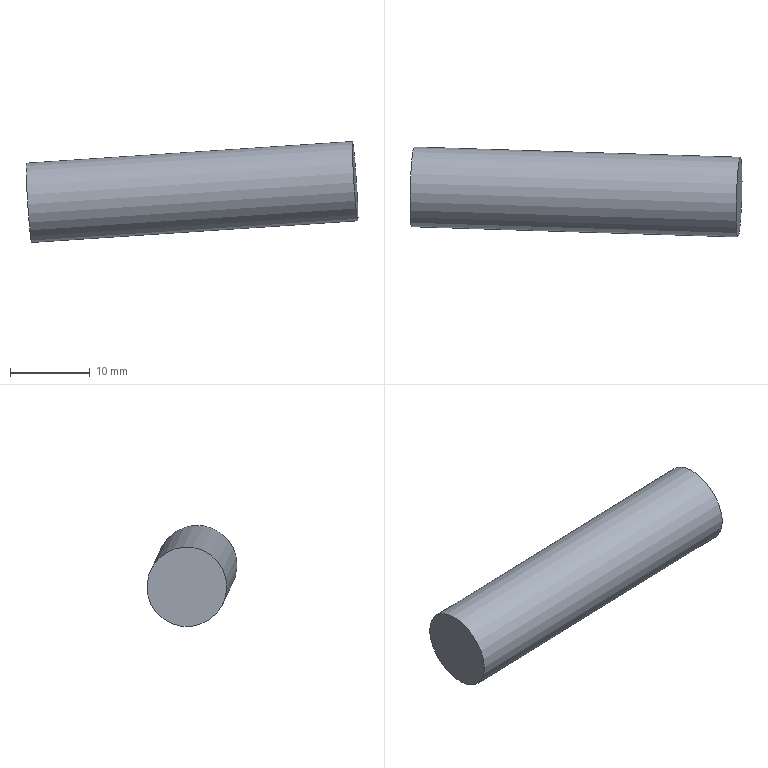Component | NX | KEY2 | 1 solid | 3 faces | box 41.62 x 11.28 x 12.69 mm | volume 3220 mm3 | plane 2 | cylinder 1 | commonest cylinder face diameters 10 x1
STEP:
#1=CARTESIAN_POINT('',(0.,0.,0.));
#2=DIRECTION('',(0.,0.,1.));
#3=DIRECTION('',(1.,0.,0.));
#4=AXIS2_PLACEMENT_3D('',#1,#2,#3);
#5=CARTESIAN_POINT('',(261.275,-324.256,279.125));
#6=VERTEX_POINT('',#5);
#7=CARTESIAN_POINT('',(261.248,-319.91,281.596));
#8=DIRECTION('',(-0.9973,0.03139,-0.06617));
#9=DIRECTION('',(0.005429,-0.8693,-0.4942));
#10=AXIS2_PLACEMENT_3D('',#7,#8,#9);
#11=CIRCLE('',#10,5.);
#12=CARTESIAN_POINT('',(261.248,-319.91,281.596));
#13=DIRECTION('',(0.9973,-0.03139,0.06617));
#14=DIRECTION('',(-0.07304,-0.4932,0.8668));
#15=AXIS2_PLACEMENT_3D('',#12,#13,#14);
#16=CYLINDRICAL_SURFACE('',#15,5.);
#17=CARTESIAN_POINT('',(7.854,0.));
#18=DIRECTION('',(-1.,0.));
#19=VECTOR('',#18,1.);
#20=LINE('',#17,#19);
#21=(GEOMETRIC_REPRESENTATION_CONTEXT(2)PARAMETRIC_REPRESENTATION_CONTEXT()REPRESENTATION_CONTEXT('',''));
#22=DEFINITIONAL_REPRESENTATION('',(#20),#21);
#23=PCURVE('',#16,#22);
#24=CARTESIAN_POINT('',(261.248,-319.91,281.596));
#25=DIRECTION('',(-0.9973,0.03139,-0.06617));
#26=DIRECTION('',(0.07304,0.4932,-0.8668));
#27=AXIS2_PLACEMENT_3D('',#24,#25,#26);
#28=PLANE('',#27);
#29=CARTESIAN_POINT('',(0.,0.));
#30=DIRECTION('',(-0.,1.));
#31=AXIS2_PLACEMENT_2D('',#29,#30);
#32=CIRCLE('',#31,5.);
#33=(GEOMETRIC_REPRESENTATION_CONTEXT(2)PARAMETRIC_REPRESENTATION_CONTEXT()REPRESENTATION_CONTEXT('',''));
#34=DEFINITIONAL_REPRESENTATION('',(#32),#33);
#35=PCURVE('',#28,#34);
#36=SURFACE_CURVE('',#11,(#23,#35),.PCURVE_S1.);
#37=EDGE_CURVE('',#6,#6,#36,.T.);
#38=ORIENTED_EDGE('',*,*,#37,.F.);
#39=CARTESIAN_POINT('',(302.165,-325.543,281.838));
#40=VERTEX_POINT('',#39);
#41=CARTESIAN_POINT('',(261.275,-324.256,279.125));
#42=CARTESIAN_POINT('',(302.165,-325.543,281.838));
#43=B_SPLINE_CURVE_WITH_KNOTS('',1,(#41,#42),.UNSPECIFIED.,.F.,.F.,(2,2),(0.,41.),.PIECEWISE_BEZIER_KNOTS.);
#44=CARTESIAN_POINT('',(7.854,0.));
#45=DIRECTION('',(0.,1.));
#46=VECTOR('',#45,1.);
#47=LINE('',#44,#46);
#48=(GEOMETRIC_REPRESENTATION_CONTEXT(2)PARAMETRIC_REPRESENTATION_CONTEXT()REPRESENTATION_CONTEXT('',''));
#49=DEFINITIONAL_REPRESENTATION('',(#47),#48);
#50=PCURVE('',#16,#49);
#51=CARTESIAN_POINT('',(1.571,0.));
#52=DIRECTION('',(0.,1.));
#53=VECTOR('',#52,1.);
#54=LINE('',#51,#53);
#55=(GEOMETRIC_REPRESENTATION_CONTEXT(2)PARAMETRIC_REPRESENTATION_CONTEXT()REPRESENTATION_CONTEXT('',''));
#56=DEFINITIONAL_REPRESENTATION('',(#54),#55);
#57=PCURVE('',#16,#56);
#58=SEAM_CURVE('',#43,(#50,#57),.PCURVE_S1.);
#59=EDGE_CURVE('',#6,#40,#58,.T.);
#60=ORIENTED_EDGE('',*,*,#59,.T.);
#61=CARTESIAN_POINT('',(302.138,-321.197,284.309));
#62=DIRECTION('',(-0.9973,0.03139,-0.06617));
#63=DIRECTION('',(0.005429,-0.8693,-0.4942));
#64=AXIS2_PLACEMENT_3D('',#61,#62,#63);
#65=CIRCLE('',#64,5.);
#66=CARTESIAN_POINT('',(7.854,41.));
#67=DIRECTION('',(-1.,0.));
#68=VECTOR('',#67,1.);
#69=LINE('',#66,#68);
#70=(GEOMETRIC_REPRESENTATION_CONTEXT(2)PARAMETRIC_REPRESENTATION_CONTEXT()REPRESENTATION_CONTEXT('',''));
#71=DEFINITIONAL_REPRESENTATION('',(#69),#70);
#72=PCURVE('',#16,#71);
#73=CARTESIAN_POINT('',(302.138,-321.197,284.309));
#74=DIRECTION('',(-0.9973,0.03139,-0.06617));
#75=DIRECTION('',(0.07304,0.4932,-0.8668));
#76=AXIS2_PLACEMENT_3D('',#73,#74,#75);
#77=PLANE('',#76);
#78=CARTESIAN_POINT('',(0.,0.));
#79=DIRECTION('',(-0.,1.));
#80=AXIS2_PLACEMENT_2D('',#78,#79);
#81=CIRCLE('',#80,5.);
#82=(GEOMETRIC_REPRESENTATION_CONTEXT(2)PARAMETRIC_REPRESENTATION_CONTEXT()REPRESENTATION_CONTEXT('',''));
#83=DEFINITIONAL_REPRESENTATION('',(#81),#82);
#84=PCURVE('',#77,#83);
#85=SURFACE_CURVE('',#65,(#72,#84),.PCURVE_S1.);
#86=EDGE_CURVE('',#40,#40,#85,.T.);
#87=ORIENTED_EDGE('',*,*,#86,.T.);
#88=ORIENTED_EDGE('',*,*,#59,.F.);
#89=EDGE_LOOP('',(#38,#60,#87,#88));
#90=FACE_BOUND('',#89,.T.);
#91=ADVANCED_FACE('',(#90),#16,.T.);
#92=ORIENTED_EDGE('',*,*,#37,.T.);
#93=EDGE_LOOP('',(#92));
#94=FACE_BOUND('',#93,.T.);
#95=ADVANCED_FACE('',(#94),#28,.T.);
#96=ORIENTED_EDGE('',*,*,#86,.F.);
#97=EDGE_LOOP('',(#96));
#98=FACE_BOUND('',#97,.T.);
#99=ADVANCED_FACE('',(#98),#77,.F.);
#100=CLOSED_SHELL('',(#91,#95,#99));
#101=MANIFOLD_SOLID_BREP('',#100);
#102=(LENGTH_UNIT()NAMED_UNIT(*)SI_UNIT(.MILLI.,.METRE.));
#103=UNCERTAINTY_MEASURE_WITH_UNIT(LENGTH_MEASURE(0.00001),#102,'','');
#104=(NAMED_UNIT(*)PLANE_ANGLE_UNIT()SI_UNIT($,.RADIAN.));
#105=(NAMED_UNIT(*)SI_UNIT($,.STERADIAN.)SOLID_ANGLE_UNIT());
#106=(GEOMETRIC_REPRESENTATION_CONTEXT(3)GLOBAL_UNCERTAINTY_ASSIGNED_CONTEXT((#103))GLOBAL_UNIT_ASSIGNED_CONTEXT((#102,#104,#105))REPRESENTATION_CONTEXT('',''));
#107=ADVANCED_BREP_SHAPE_REPRESENTATION('',(#4,#101),#106);